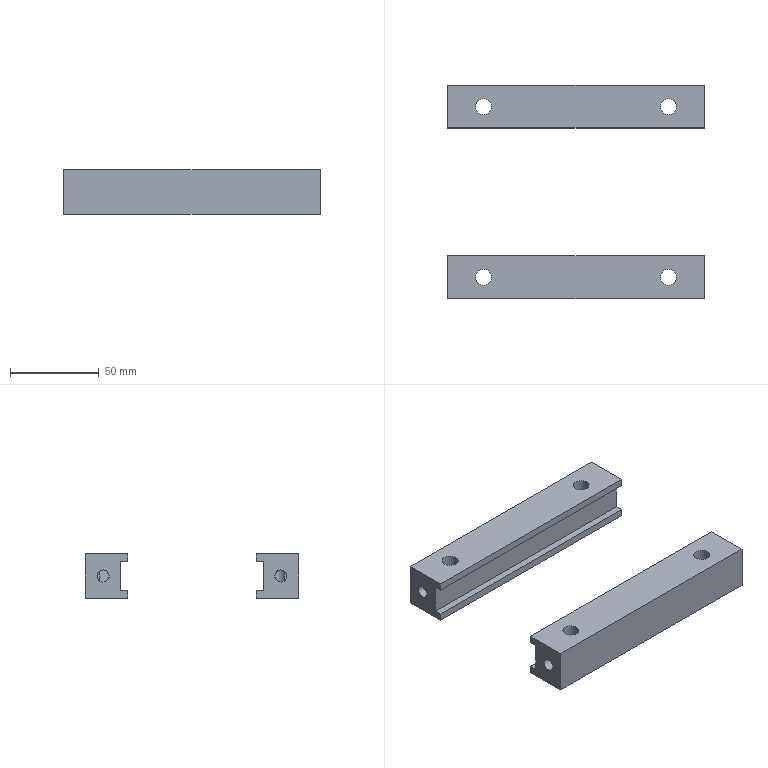Component | NX | FIXTURE | 2 solids | 40 faces | volume 142090 mm3 | plane 28 | cylinder 12 | commonest cylinder face diameters 9 x4 6.8 x4 14 x4